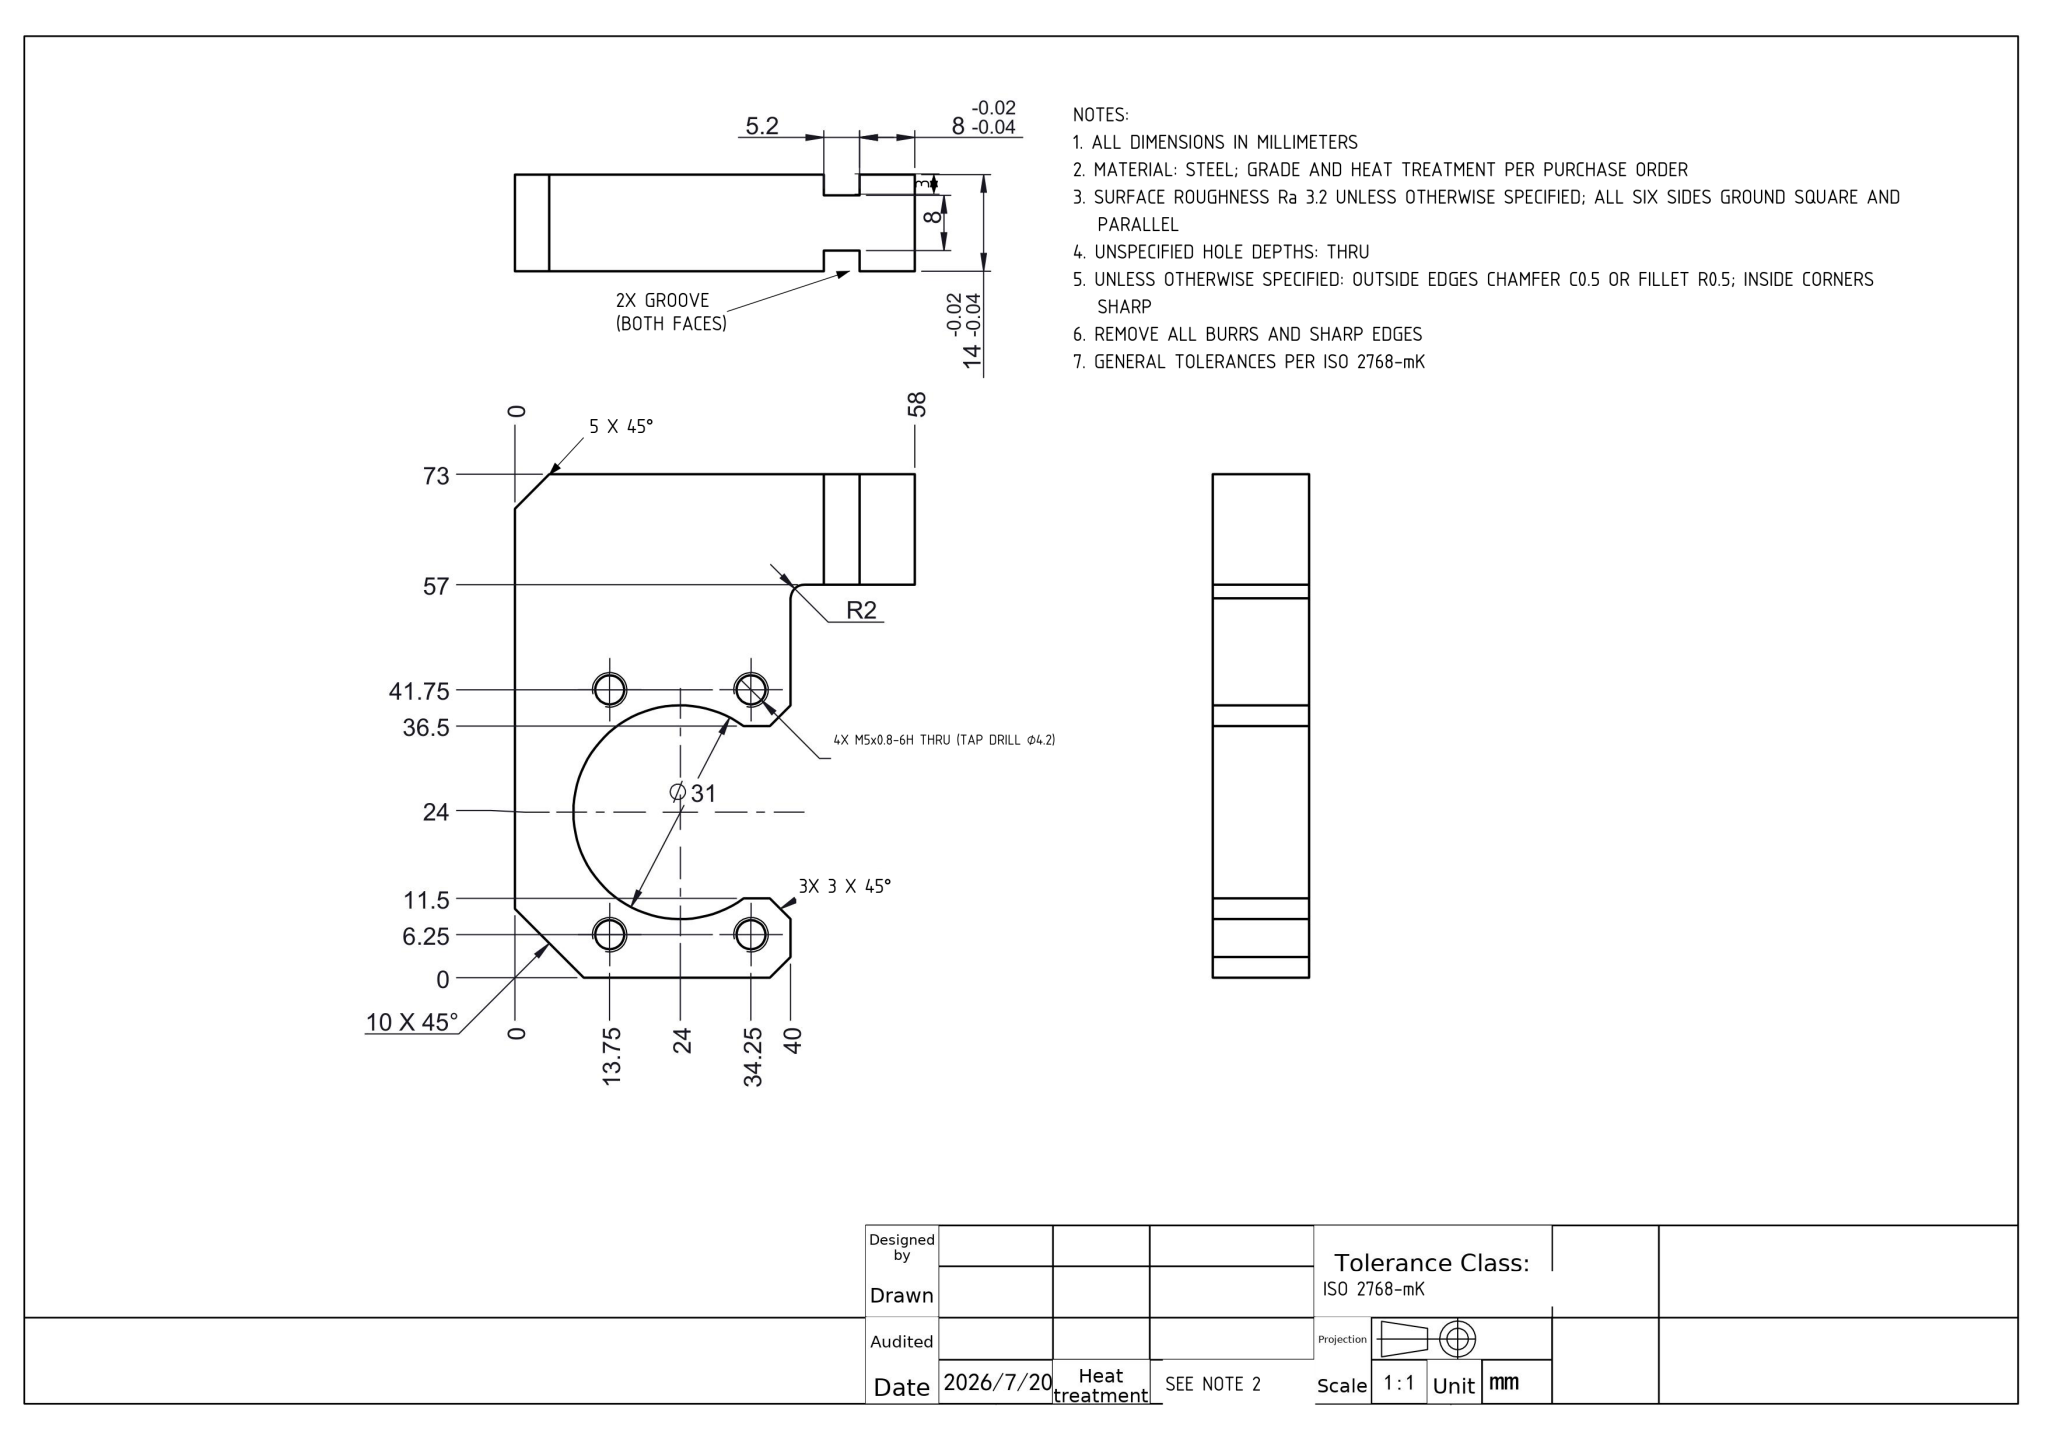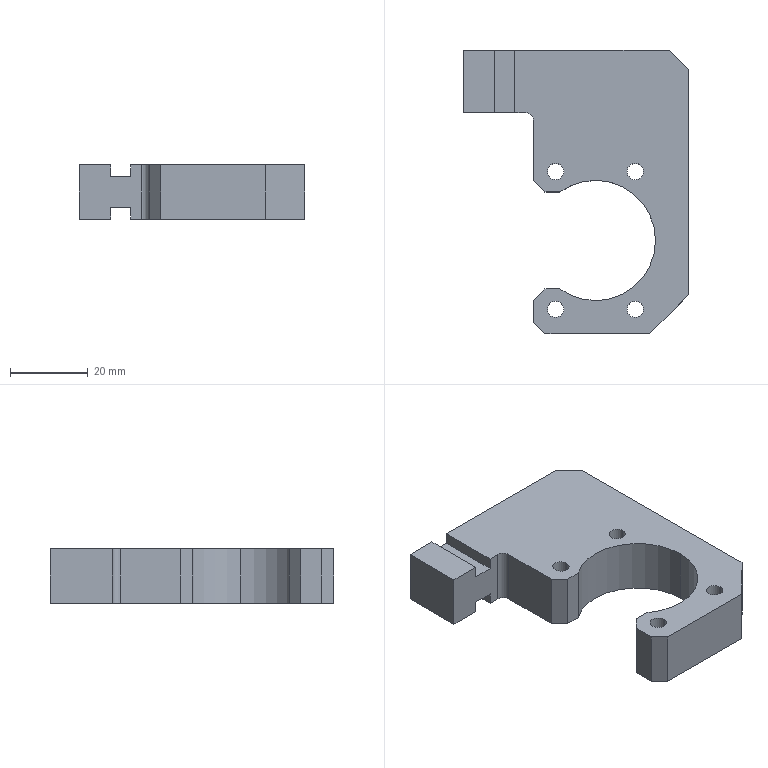Part | NX | mm | 1 solid | 35 faces | box 58 x 73 x 14 mm | volume 31178 mm3 | plane 24 | cylinder 11 | commonest cylinder face diameters 4.2 x8 31 x2 4 x1